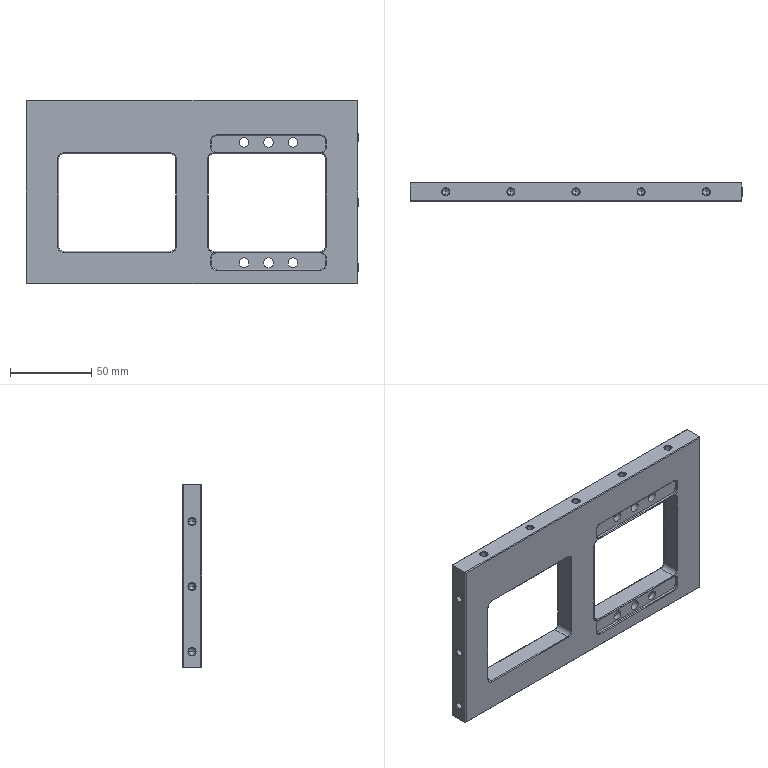Component | SolidWorks | Z-AxisElectricScrewdriverBasePlate-1 | 1 solid | 198 faces | volume 164752 mm3 | cylinder 90 | cone 44 | torus 36 | plane 28 | commonest cylinder face diameters 1 x32 6 x28 4.2 x22 11 x8